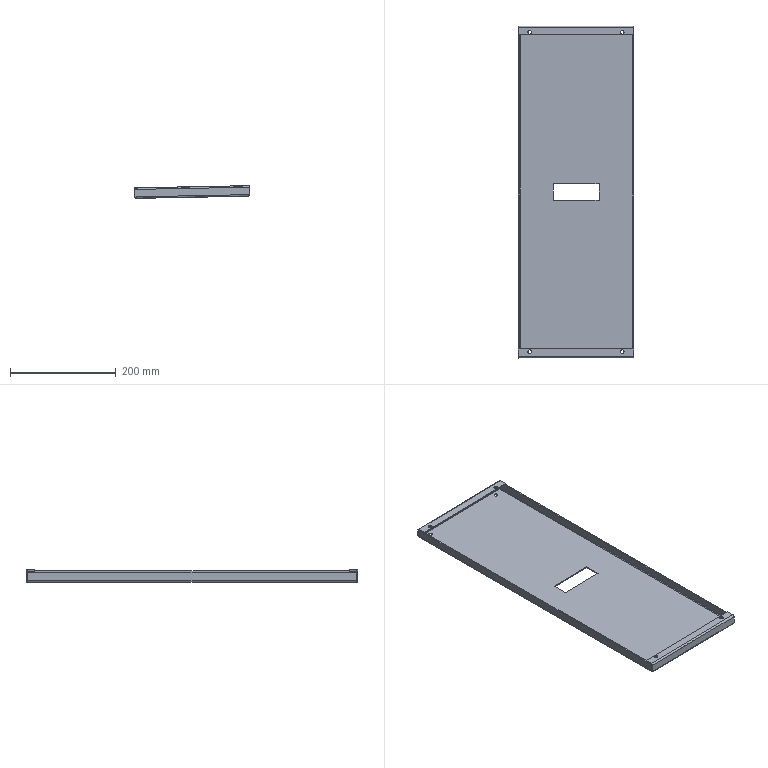Component | SolidWorks | 03FrameEndPlate2-2 | 1 solid | 78 faces | volume 332512 mm3 | plane 50 | cylinder 28 | commonest cylinder face diameters 7 x16 6 x6 2 x6 | material A3 Steel